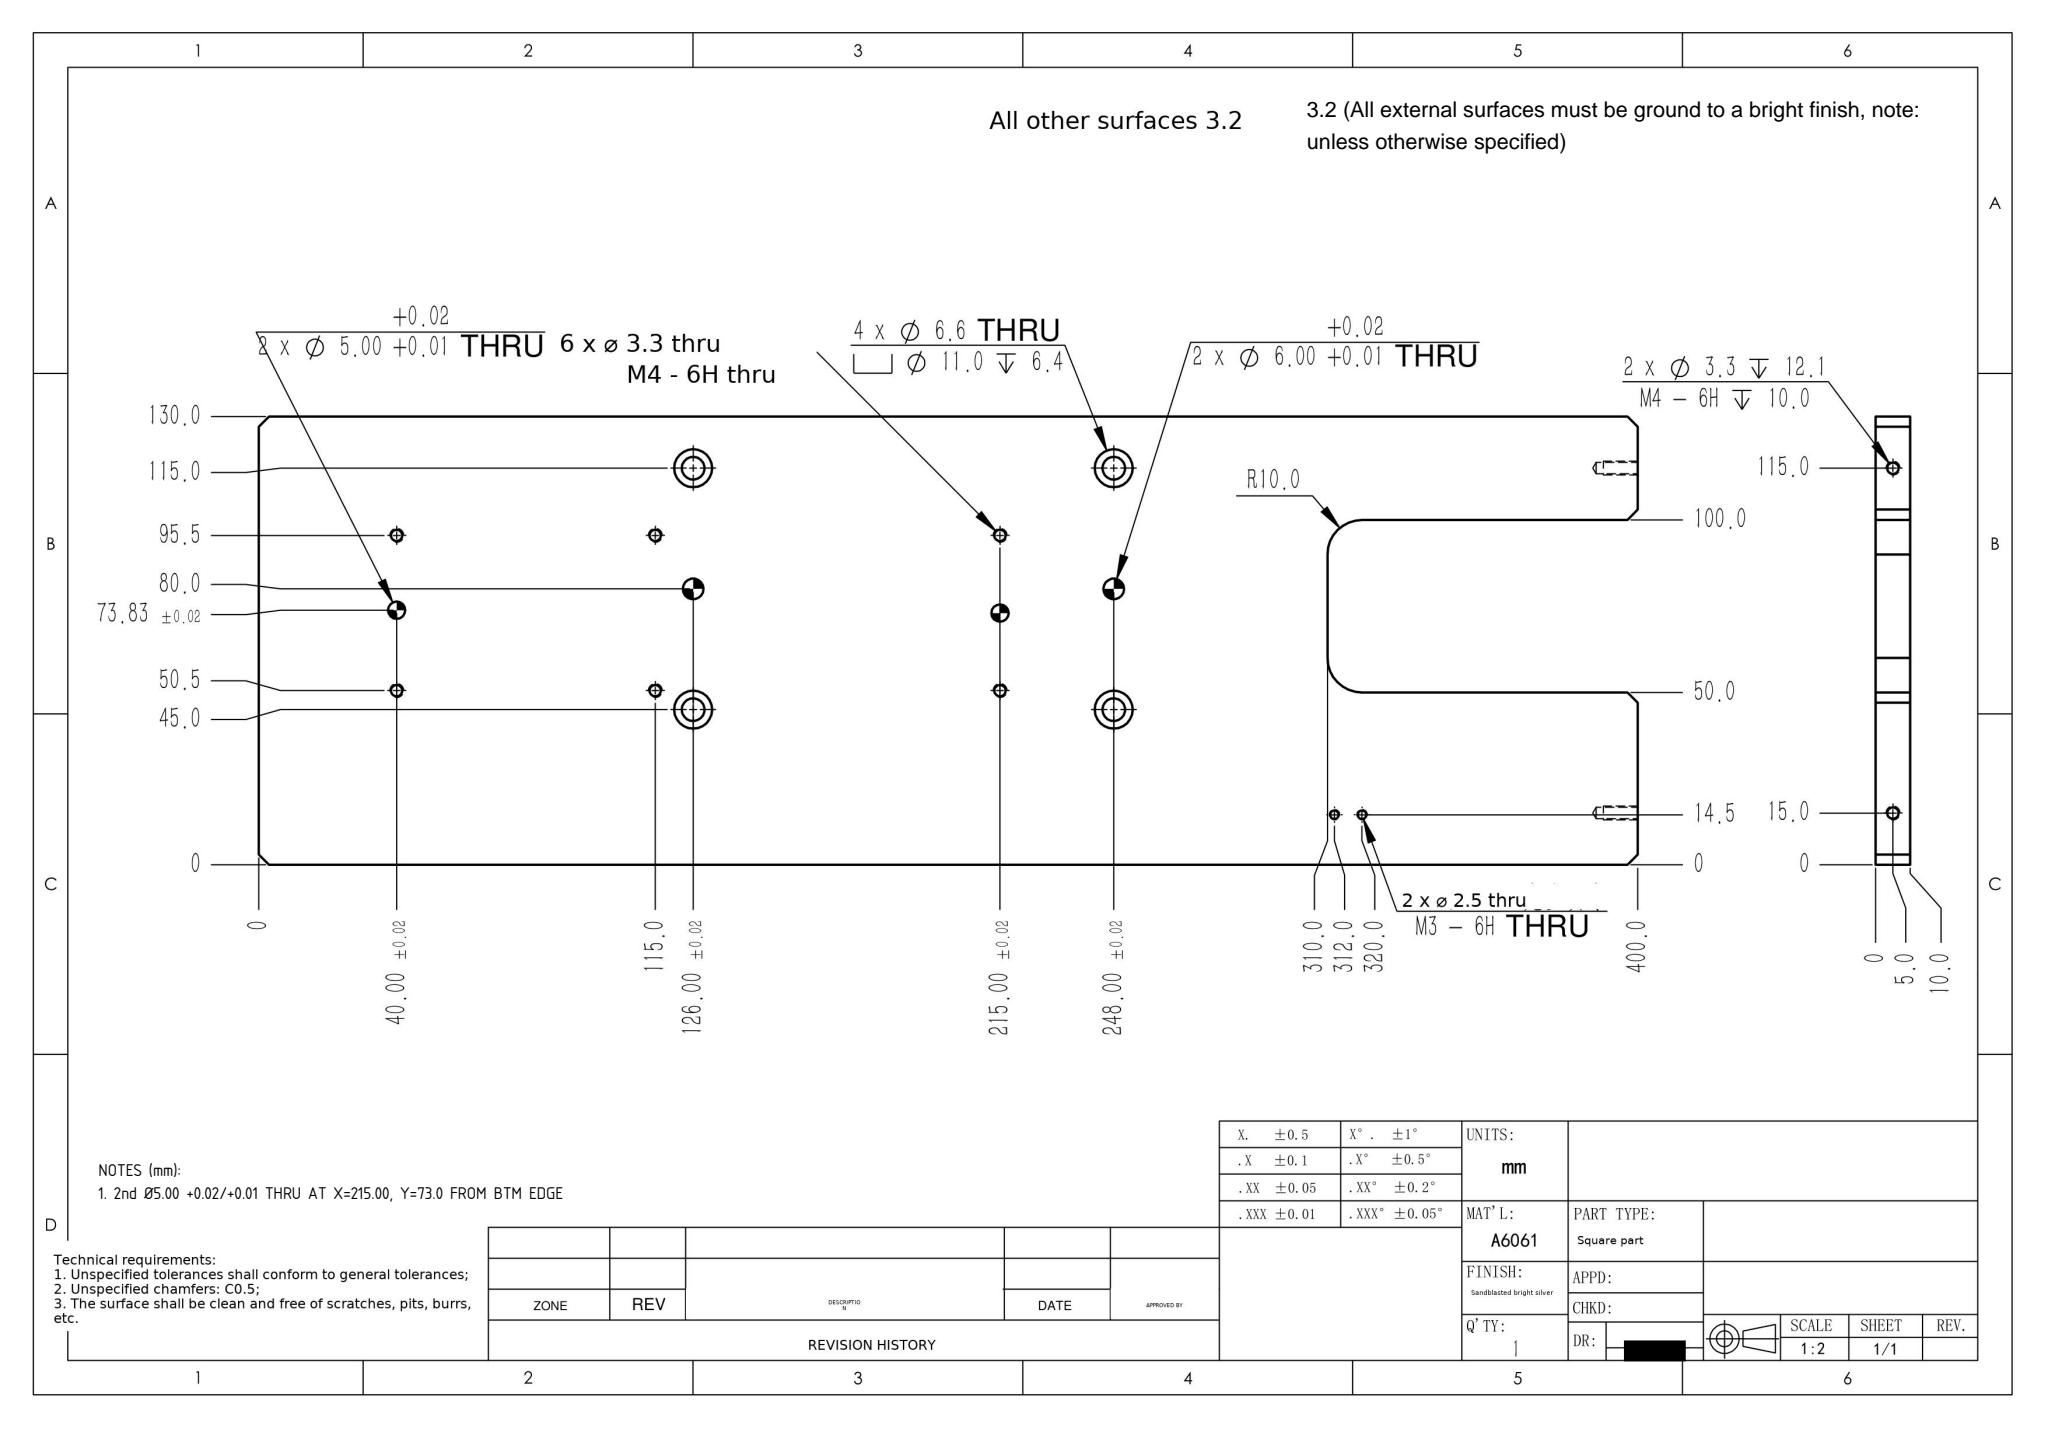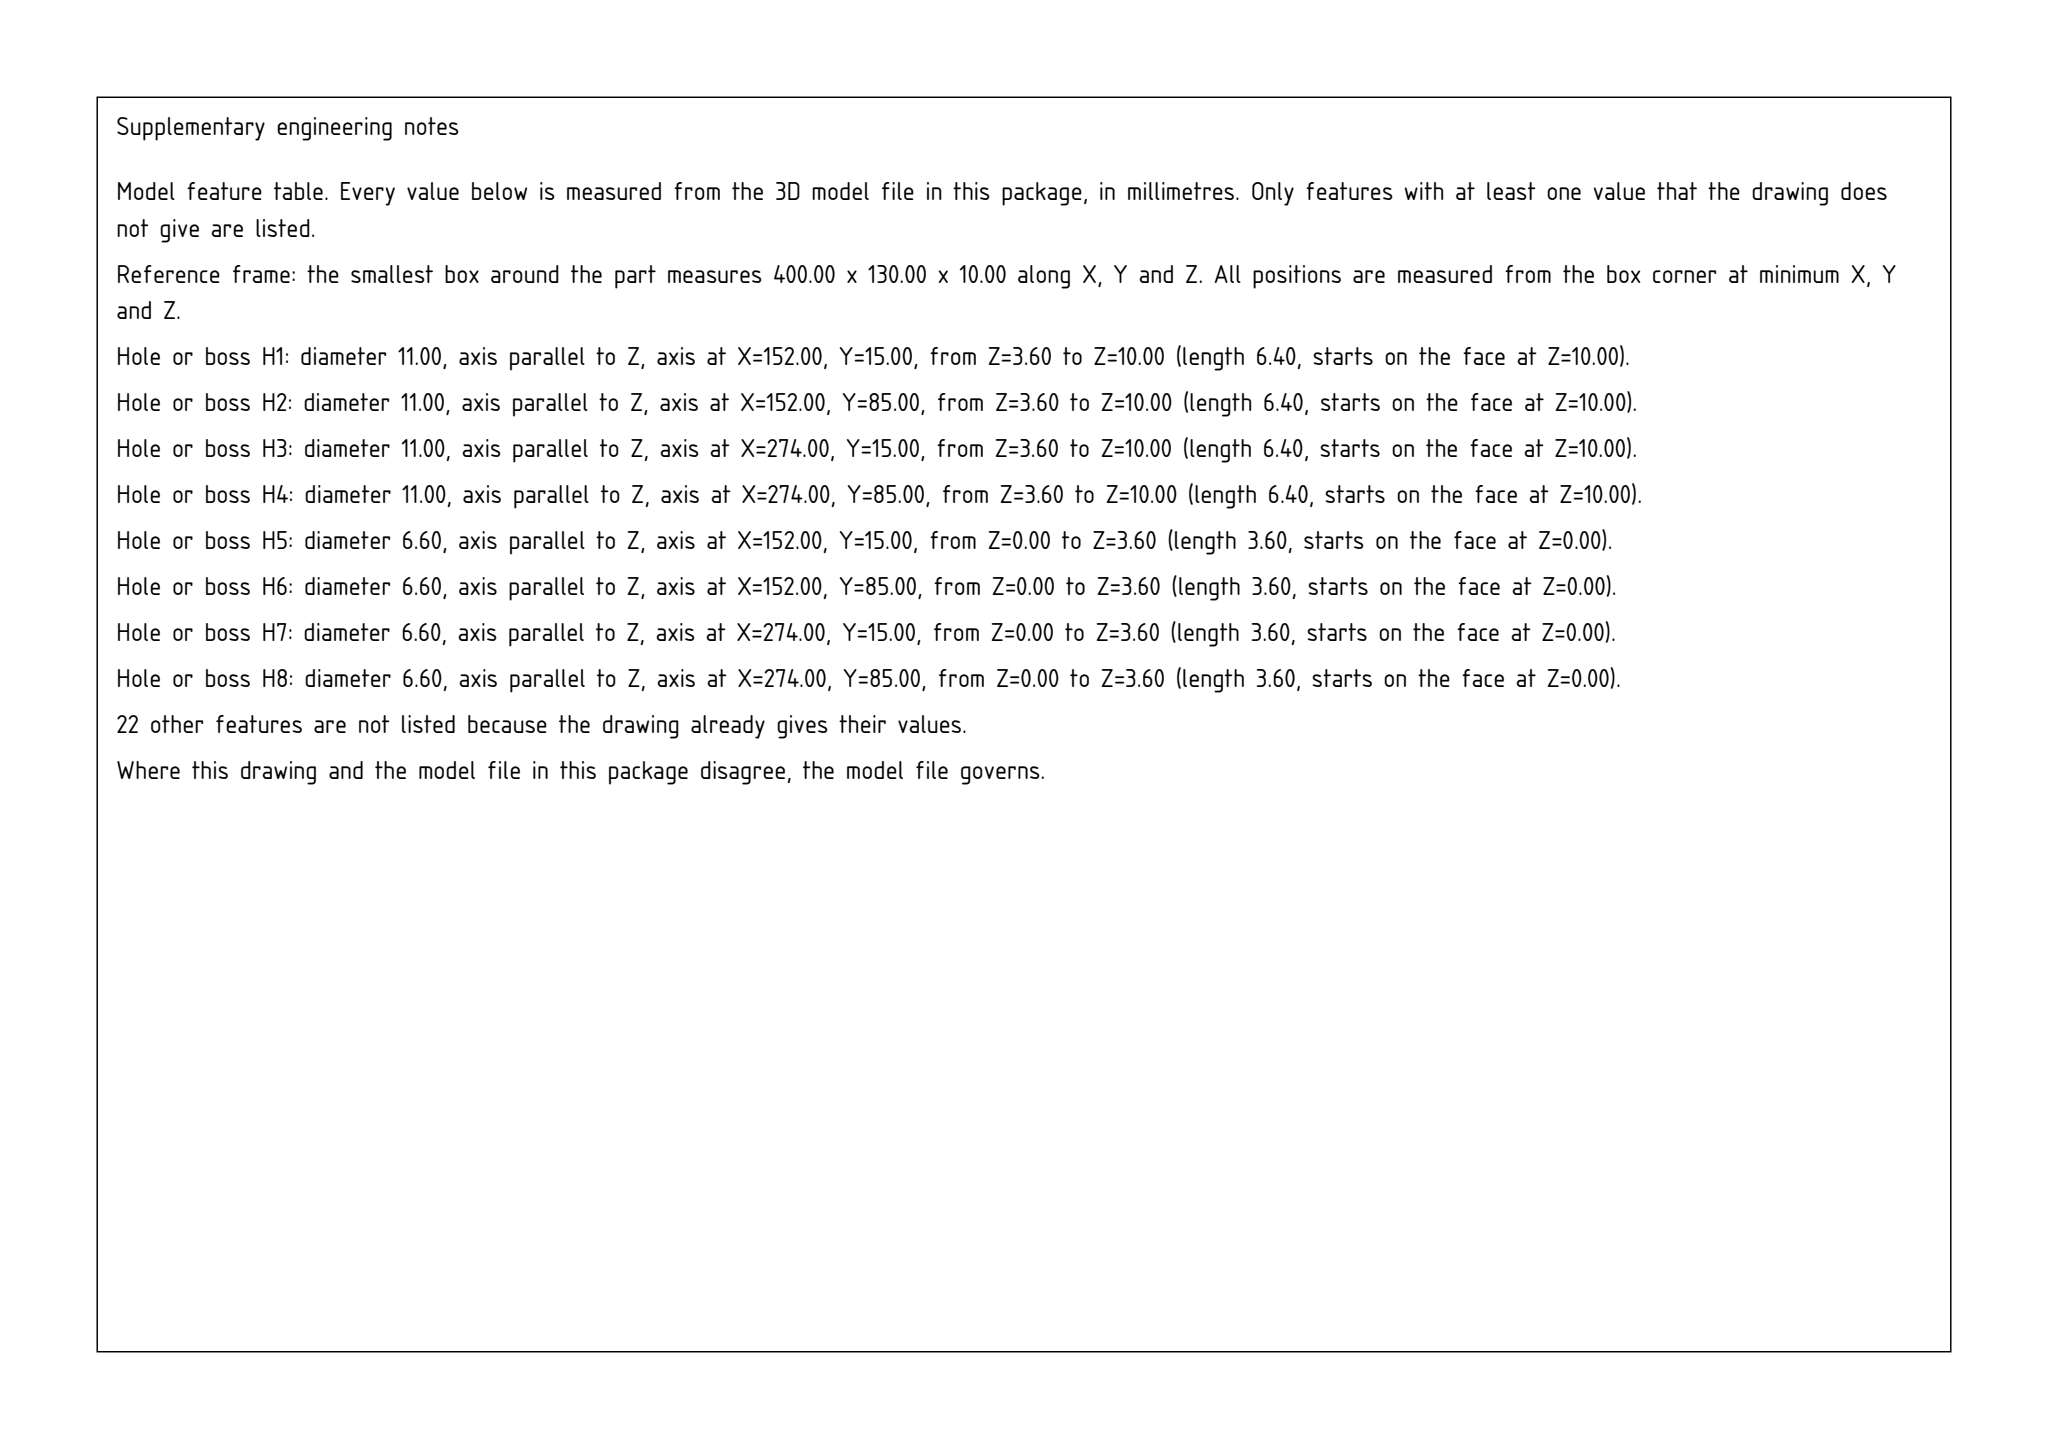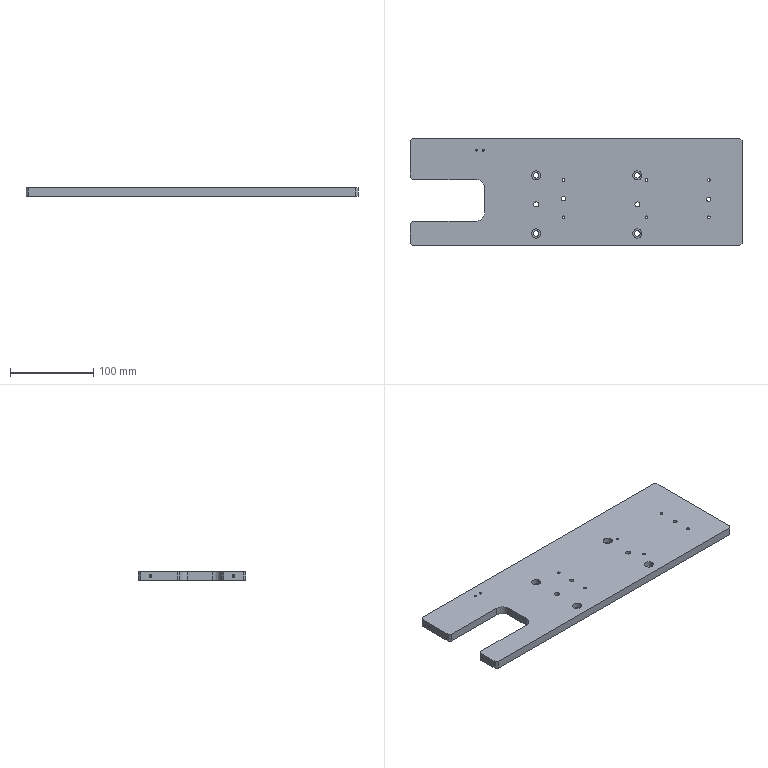Part | SolidWorks | mm | 1 solid | 70 faces | box 400 x 130 x 10 mm | volume 470452 mm3 | cylinder 46 | plane 20 | cone 4 | commonest cylinder face diameters 3.3 x16 11 x8 6.6 x8 5 x4 6 x4 2.5 x4 20 x2
Drawing notes:
2nd Ø5.00 +0.02/+0.01 THRU AT X=215.00, Y=73.0 FROM BTM EDGE | from the solid: Ø5.0 z-cyl axis at (185.0,57.0); drawing X=400-185=215.00, Y=130-57.0=73.0
build123d program:
from build123d import *

# Parameters (mm, degrees)
SKETCH1_W                                       = 400
SKETCH1_H                                       = 130
BOSS_EXTRUDE1_DEPTH                             = 10
SKETCH12_W                                      = 90
SKETCH12_H                                      = 50
CUT_EXTRUDE1_DEPTH                              = 211.535
M6_HEX_SOCKET_HEAD_CAP_SCREW_CBORE1_D           = 6.6
M6_HEX_SOCKET_HEAD_CAP_SCREW_CBORE1_CBORE_D     = 11
M6_HEX_SOCKET_HEAD_CAP_SCREW_CBORE1_CBORE_DEPTH = 6.4
M3_TAPPED_HOLE1_D                               = 2.5
M4_TAPPED_HOLE2_D                               = 3.3
SIZE_MM_DOWEL_HOLE1_D                           = 6
M4_TAPPED_HOLE3_D                               = 3.3
M4_TAPPED_HOLE3_DEPTH                           = 12.1
M4_TAPPED_HOLE3_TIP                             = 0.9914
SIZE_MM_DOWEL_HOLE2_D                           = 5
FILLET1_R                                       = 10
CHAMFER1_SIZE                                   = 3


with BuildPart() as part:
    # Sketch1 → Boss-Extrude1 (new body)
    with BuildSketch(Plane.XY):
        Rectangle(SKETCH1_W, SKETCH1_H)
    extrude(amount=BOSS_EXTRUDE1_DEPTH)

    # Sketch12 → Cut-Extrude1 (cut, through all)
    with BuildSketch(Plane.XY.offset(10)):
        with Locations((-155, -10)):
            Rectangle(SKETCH12_W, SKETCH12_H)
    extrude(amount=-CUT_EXTRUDE1_DEPTH, mode=Mode.SUBTRACT)

    # M6 Hex Socket Head Cap Screw CBORE1 (through all)
    with Locations(Plane.XY.offset(10)):
        with Locations((-48, -50), (-48, 20), (74, 20), (74, -50)):
            CounterBoreHole(M6_HEX_SOCKET_HEAD_CAP_SCREW_CBORE1_D / 2, M6_HEX_SOCKET_HEAD_CAP_SCREW_CBORE1_CBORE_D / 2, M6_HEX_SOCKET_HEAD_CAP_SCREW_CBORE1_CBORE_DEPTH)

    # M3 Tapped Hole1 (through all)
    with Locations(Plane.XY.offset(10)):
        with Locations((-120, 50.5), (-112, 50.5)):
            Hole(M3_TAPPED_HOLE1_D / 2)

    # M4 Tapped Hole2 (through all)
    with Locations(Plane.XY.offset(10)):
        with Locations((-15, 14.5), (85, 14.5), (160, 14.5), (160, -30.5), (85, -30.5), (-15, -30.5)):
            Hole(M4_TAPPED_HOLE2_D / 2)

    # Size mm Dowel Hole1 (through all)
    with Locations(Plane.XY.offset(10)):
        with Locations((-48, -15), (74, -15)):
            Hole(SIZE_MM_DOWEL_HOLE1_D / 2)

    # M4 Tapped Hole3
    with Locations(Plane.ZY.offset(200)):
        with Locations((5, -50), (5, 50)):
            Hole(M4_TAPPED_HOLE3_D / 2, depth=M4_TAPPED_HOLE3_DEPTH)
            with Locations((0, 0, -(M4_TAPPED_HOLE3_DEPTH + M4_TAPPED_HOLE3_TIP / 2))):  # 118° drill point
                Cone(0, M4_TAPPED_HOLE3_D / 2, M4_TAPPED_HOLE3_TIP, mode=Mode.SUBTRACT)

    # Size mm Dowel Hole2 (through all)
    with Locations(Plane.XY.offset(10)):
        with Locations((160, -8.825), (-15, -8)):
            Hole(SIZE_MM_DOWEL_HOLE2_D / 2)

    # Fillet1
    fillet1_edges = [part.edges().sort_by_distance(p)[0] for p in [
        (-110, 15, 5),
        (-110, -35, 5),
    ]]
    fillet(fillet1_edges, radius=FILLET1_R)

    # Chamfer1
    chamfer1_edges = [part.edges().sort_by_distance(p)[0] for p in [
        (-200, -35, 5),
        (-200, 15, 5),
        (200, -65, 5),
        (-200, -65, 5),
        (-200, 65, 5),
        (200, 65, 5),
    ]]
    chamfer(chamfer1_edges, length=CHAMFER1_SIZE)


solid = part.part